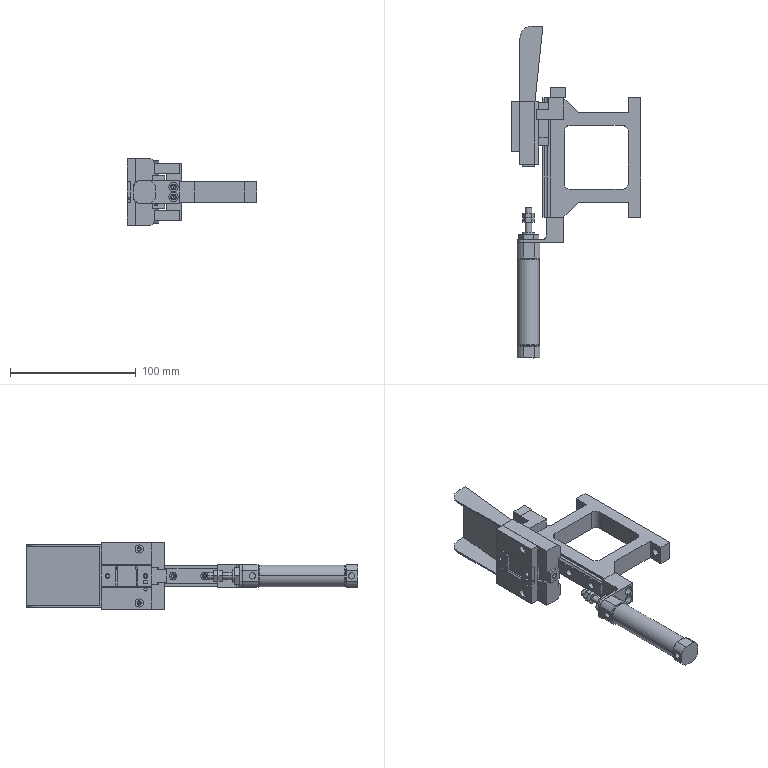Assembly | SolidWorks | mm | 14 component files | 14 solids | 618 faces | box 103.3 x 264 x 53 mm | volume 155353 mm3 | plane 338 | cylinder 180 | spline 52 | cone 48 | commonest cylinder face diameters 2.5 x24 3.3 x16 4.5 x16 6 x13 3.5 x12 6.5 x12 3.4 x12 10 x10
Bill of materials:
7.1.02.0001.00.00-0049 | 1 |  | Flat rectangular frame plate with a large rounded-rectangle through-window and an H-like outline formed by notches cut into two opposite sides.
7.1.02.0001.00.00-0050 | 1 |  | L-shaped bracket: a thin plate with a rounded end and a large through-hole, joined to a thicker rectangular block that has two smaller parallel through-holes.
7.1.02.0001.00.00-0052 | 1 |  | Rectangular block with a stepped profile, giving a raised tongue or T-shaped section, and one round through-hole across the block.
7.1.02.0001.00.00-0053 | 1 |  | Rectangular bar with four round through-holes in a straight line: two larger holes near the ends and two smaller holes near the middle.
7.1.02.0001.00.00-0054 | 2 |  | Solid L-shaped prism block with no holes or other features.
7.1.02.0001.00.00-0055 | 1 |  | Thick plate with a wedge-shaped (tapered) cross-section and a rounded edge at the thicker end; two small holes in one narrow end face.
7.1.02.0001.00.00-0081 | 1 |  | Rectangular machined plate with chamfered edges, a rectangular notch in one side, stepped grooves or rebates, and six round through-holes in two sizes.
7.1.02.0001.00.00-0082 | 1 |  | Rectangular plate with a raised rib across the middle of one face, recessed or chamfered shoulders on the opposite face, six round holes and two small slots.
7.1.02.0001.00.00-0083 | 1 |  | Rectangular plate with a stepped corner notch and a chamfered edge, a large round through-hole, a rectangular through-window, and a small hole in one side edge.
7.1.02.0001.00.00-0084 | 1 |  | Rectangular plate with a stepped corner notch, a chamfered edge, a shallow rebate along one face, and one round through-hole.
AB16X45 | 1 |  | Long cylindrical body with end caps that are square with chamfered corners at both ends, and a smaller rod coming out of one end with hex-shaped nut features and a reduced-diameter tip.
MGN12C-ElectricalTestFailureExclusionGuideRail | 1 |  | Long prismatic rail with a roughly rectangular section, chamfered corners, two semicircular grooves running lengthwise on opposite faces, and a row of four evenly spaced holes through the side.
MGN12C-ElectricalTestFailureExclusionSlider | 1 |  | Simplified rectangular block with a C-shaped channel running its full length and open on one side. Each inner corner of the channel has a semicircular groove; a half-round bead runs the length of one of them. The block has a stepped outer profile: the middle section along its length sits slightly proud of the two end sections. One end face has a small round hole and engraved text. The overall shape looks like a linear-guide carriage, but this is not confirmed.
Mates:
1. concentric | 7.1.02.0001.00.00-0049-1 face at (-30.964, -48.684, 4) dir (0, -1, 0) r 1.65 | 7.1.02.0001.00.00-0050-1 face at (-30.964, -68.684, 4) dir (0, -1, 0) r 2.25
2. concentric | 7.1.02.0001.00.00-0049-1 face at (-30.964, -48.684, -4) dir (0, -1, 0) r 1.65 | 7.1.02.0001.00.00-0050-1 face at (-30.964, -68.684, -4) dir (0, -1, 0) r 2.25
3. coincident | 7.1.02.0001.00.00-0049-1 face at (-36.964, -48.684, 8) dir (0, -1, 0) | 7.1.02.0001.00.00-0050-1 face at (-39.964, -48.684, -9) dir (0, 1, 0)
4. concentric | 7.1.02.0001.00.00-0049-1 face at (-30.964, 46.316, -4) dir (0, 1, 0) r 1.65 | 7.1.02.0001.00.00-0053-1 face at (-30.964, 54.316, -4) dir (0, -1, 0) r 2.25
5. concentric | 7.1.02.0001.00.00-0049-1 face at (-30.964, 46.316, 4) dir (0, 1, 0) r 1.65 | 7.1.02.0001.00.00-0053-1 face at (-30.964, 54.316, 4) dir (0, -1, 0) r 2.25
6. coincident | 7.1.02.0001.00.00-0049-1 face at (-36.964, 46.316, 8) dir (0, 1, 0) | 7.1.02.0001.00.00-0053-1 face at (-30.964, 46.316, 0) dir (0, -1, 0)
7. concentric | 7.1.02.0001.00.00-0049-1 face at (-34.964, -38.684, 0) dir (-1, 0, 0) r 1.25 | ElectricalTestFailureExclusionLinearGuideMGN12C1R95Z0M-1/MGN12C-ElectricalTestFailureExclusionGuideRail-1 face at (-25.987, -38.684, 0) dir (1, 0, 0) r 1.75
8. concentric | 7.1.02.0001.00.00-0049-1 face at (-34.964, 36.316, 0) dir (-1, 0, 0) r 1.25 | ElectricalTestFailureExclusionLinearGuideMGN12C1R95Z0M-1/MGN12C-ElectricalTestFailureExclusionGuideRail-1 face at (-42.964, 36.316, 0) dir (-1, 0, 0) r 1.75
9. coincident | 7.1.02.0001.00.00-0049-1 face at (-34.964, 46.316, 6) dir (-1, 0, 0) | ElectricalTestFailureExclusionLinearGuideMGN12C1R95Z0M-1/MGN12C-ElectricalTestFailureExclusionGuideRail-1 face at (-34.964, 21.316, 6) dir (1, 0, 0)
10. concentric | ElectricalTestFailureExclusionLinearGuideMGN12C1R95Z0M-1/MGN12C-ElectricalTestFailureExclusionSlider-1 face at (-47.964, 32.916, -10) dir (1, 0, 0) r 1.5 | 7.1.02.0001.00.00-0081-1 face at (-60.964, 32.916, -10) dir (-1, 0, 0) r 1.7
11. concentric | ElectricalTestFailureExclusionLinearGuideMGN12C1R95Z0M-1/MGN12C-ElectricalTestFailureExclusionSlider-1 face at (-47.964, 17.916, 10) dir (1, 0, 0) r 1.5 | 7.1.02.0001.00.00-0081-1 face at (-60.964, 17.916, 10) dir (-1, 0, 0) r 1.7
12. coincident | ElectricalTestFailureExclusionLinearGuideMGN12C1R95Z0M-1/MGN12C-ElectricalTestFailureExclusionSlider-1 face at (-47.964, 42.766, 13.5) dir (-1, 0, 0) | 7.1.02.0001.00.00-0081-1 face at (-47.964, -6.684, 13.5) dir (1, 0, 0)
13. concentric | 7.1.02.0001.00.00-0081-1 face at (-60.964, 32.916, 18.5) dir (-1, 0, 0) r 2.25 | 7.1.02.0001.00.00-0054-1 face at (-47.964, 32.916, 18.5) dir (-1, 0, 0) r 1.65
14. coincident | 7.1.02.0001.00.00-0081-1 face at (-47.964, -6.684, 13.5) dir (1, 0, 0) | 7.1.02.0001.00.00-0054-1 face at (-47.964, 28.916, 14.5) dir (-1, 0, 0)
15. parallel | 7.1.02.0001.00.00-0081-1 face at (-60.964, -6.684, 26.5) dir (0, 0, 1) | 7.1.02.0001.00.00-0054-1 face at (-36.964, 37.616, 22.5) dir (0, 0, 1)
16. concentric | 7.1.02.0001.00.00-0081-1 face at (-60.964, 32.916, -18.5) dir (-1, 0, 0) r 2.25 | 7.1.02.0001.00.00-0054-2 face at (-47.964, 32.916, -18.5) dir (-1, 0, 0) r 1.65
17. coincident | 7.1.02.0001.00.00-0081-1 face at (-47.964, -6.684, 13.5) dir (1, 0, 0) | 7.1.02.0001.00.00-0054-2 face at (-47.964, 28.916, -22.5) dir (-1, 0, 0)
18. parallel | 7.1.02.0001.00.00-0081-1 face at (-60.964, -6.684, -26.5) dir (0, 0, -1) | 7.1.02.0001.00.00-0054-2 face at (-36.964, 37.616, -22.5) dir (0, 0, -1)
19. distance | 7.1.02.0001.00.00-0054-2 face at (-37.964, 46.316, -22.5) dir (0, 1, 0) | 7.1.02.0001.00.00-0053-1 face at (-30.964, 46.316, 0) dir (0, -1, 0)
20. concentric | 7.1.02.0001.00.00-0081-1 face at (-54.464, 43.316, -4) dir (0, 1, 0) r 1.65 | 7.1.02.0001.00.00-0055-1 face at (-54.464, 103.316, -4) dir (0, -1, 0) r 2.25
21. concentric | 7.1.02.0001.00.00-0081-1 face at (-54.464, 43.316, 4) dir (0, 1, 0) r 1.65 | 7.1.02.0001.00.00-0055-1 face at (-54.464, 103.316, 4) dir (0, -1, 0) r 2.25
22. coincident | 7.1.02.0001.00.00-0081-1 face at (-60.964, 43.316, 26.5) dir (0, 1, 0) | 7.1.02.0001.00.00-0055-1 face at (-60.964, 43.316, -25) dir (0, -1, 0)
23. concentric | 7.1.02.0001.00.00-0050-1 face at (-54.064, -48.684, 0) dir (0, -1, 0) r 5.25 | AB16X45-1 face at (-54.064, -64.934, 0) dir (0, 1, 0) r 5
24. coincident | 7.1.02.0001.00.00-0050-1 face at (-63.064, -68.684, -9) dir (0, -1, 0) | AB16X45-1 face at (-47.064, -68.684, -0.05897) dir (0, 1, 0)
25. concentric | 7.1.02.0001.00.00-0052-1 face at (-54.064, -8.684, 0) dir (0, -1, 0) r 2.1 | AB16X45-1 face at (-54.064, -50.934, 0) dir (0, 1, 0) r 2.5
26. coincident | 7.1.02.0001.00.00-0081-1 face at (-60.964, 3.316, 7.1) dir (0, -1, 0) | 7.1.02.0001.00.00-0052-1 face at (-59.064, 3.316, 7) dir (0, 1, 0)
27. parallel | 7.1.02.0001.00.00-0081-1 face at (-60.964, 18.316, 0) dir (-1, 0, 0) | 7.1.02.0001.00.00-0052-1 face at (-59.064, -2.684, 0) dir (-1, 0, 0)
28. concentric | 7.1.02.0001.00.00-0081-1 face at (-60.964, 13.316, -21.5) dir (-1, 0, 0) r 1.25 | 7.1.02.0001.00.00-0082-1 face at (-67.964, 13.316, -21.5) dir (-1, 0, 0) r 1.7
29. concentric | 7.1.02.0001.00.00-0081-1 face at (-60.964, 13.316, 21.5) dir (-1, 0, 0) r 1.25 | 7.1.02.0001.00.00-0082-1 face at (-67.964, 13.316, 21.5) dir (-1, 0, 0) r 1.7
30. coincident | 7.1.02.0001.00.00-0081-1 face at (-60.964, 18.316, 0) dir (-1, 0, 0) | 7.1.02.0001.00.00-0082-1 face at (-60.964, 23.316, 0) dir (1, 0, 0)
31. concentric | 7.1.02.0001.00.00-0082-1 face at (-65.164, 8.316, 0) dir (-1, 0, 0) r 1.25 | 7.1.02.0001.00.00-0083-1 face at (-65.164, 8.316, 0) dir (-1, 0, 0) r 1.75
32. parallel | 7.1.02.0001.00.00-0082-1 face at (-67.964, 3.316, -26.5) dir (0, -1, 0) | 7.1.02.0001.00.00-0083-1 face at (-65.164, 3.316, 8.05) dir (0, -1, 0)
33. coincident | 7.1.02.0001.00.00-0082-1 face at (-65.164, 43.316, -8.1) dir (-1, 0, 0) | 7.1.02.0001.00.00-0083-1 face at (-65.164, 9.491, 0) dir (1, 0, 0)
34. concentric | 7.1.02.0001.00.00-0082-1 face at (-65.164, 38.316, 0) dir (-1, 0, 0) r 1.25 | 7.1.02.0001.00.00-0084-1 face at (-65.164, 38.316, 0) dir (-1, 0, 0) r 1.75
35. coincident | 7.1.02.0001.00.00-0082-1 face at (-65.164, 43.316, -8.1) dir (-1, 0, 0) | 7.1.02.0001.00.00-0084-1 face at (-65.164, 37.141, 0) dir (1, 0, 0)
36. parallel | 7.1.02.0001.00.00-0082-1 face at (-67.964, 43.316, -26.5) dir (0, 1, 0) | 7.1.02.0001.00.00-0084-1 face at (-65.164, 43.316, -8.05) dir (0, 1, 0)
37. coincident | MGN12C-ElectricalTestFailureExclusionGuideRail-1 face at (1.516, 8.101, 34.619) dir (0, 1, 0) | MGN12C-ElectricalTestFailureExclusionSlider-1 face at (1.516, 8.101, 73.719) dir (0, -1, 0)
38. concentric | MGN12C-ElectricalTestFailureExclusionGuideRail-1 face at (1.516, 5.601, 34.619) dir (0, 0, -1) r 1.25 | MGN12C-ElectricalTestFailureExclusionSlider-1 face at (1.516, 5.601, 73.719) dir (0, 0, -1) r 1.25